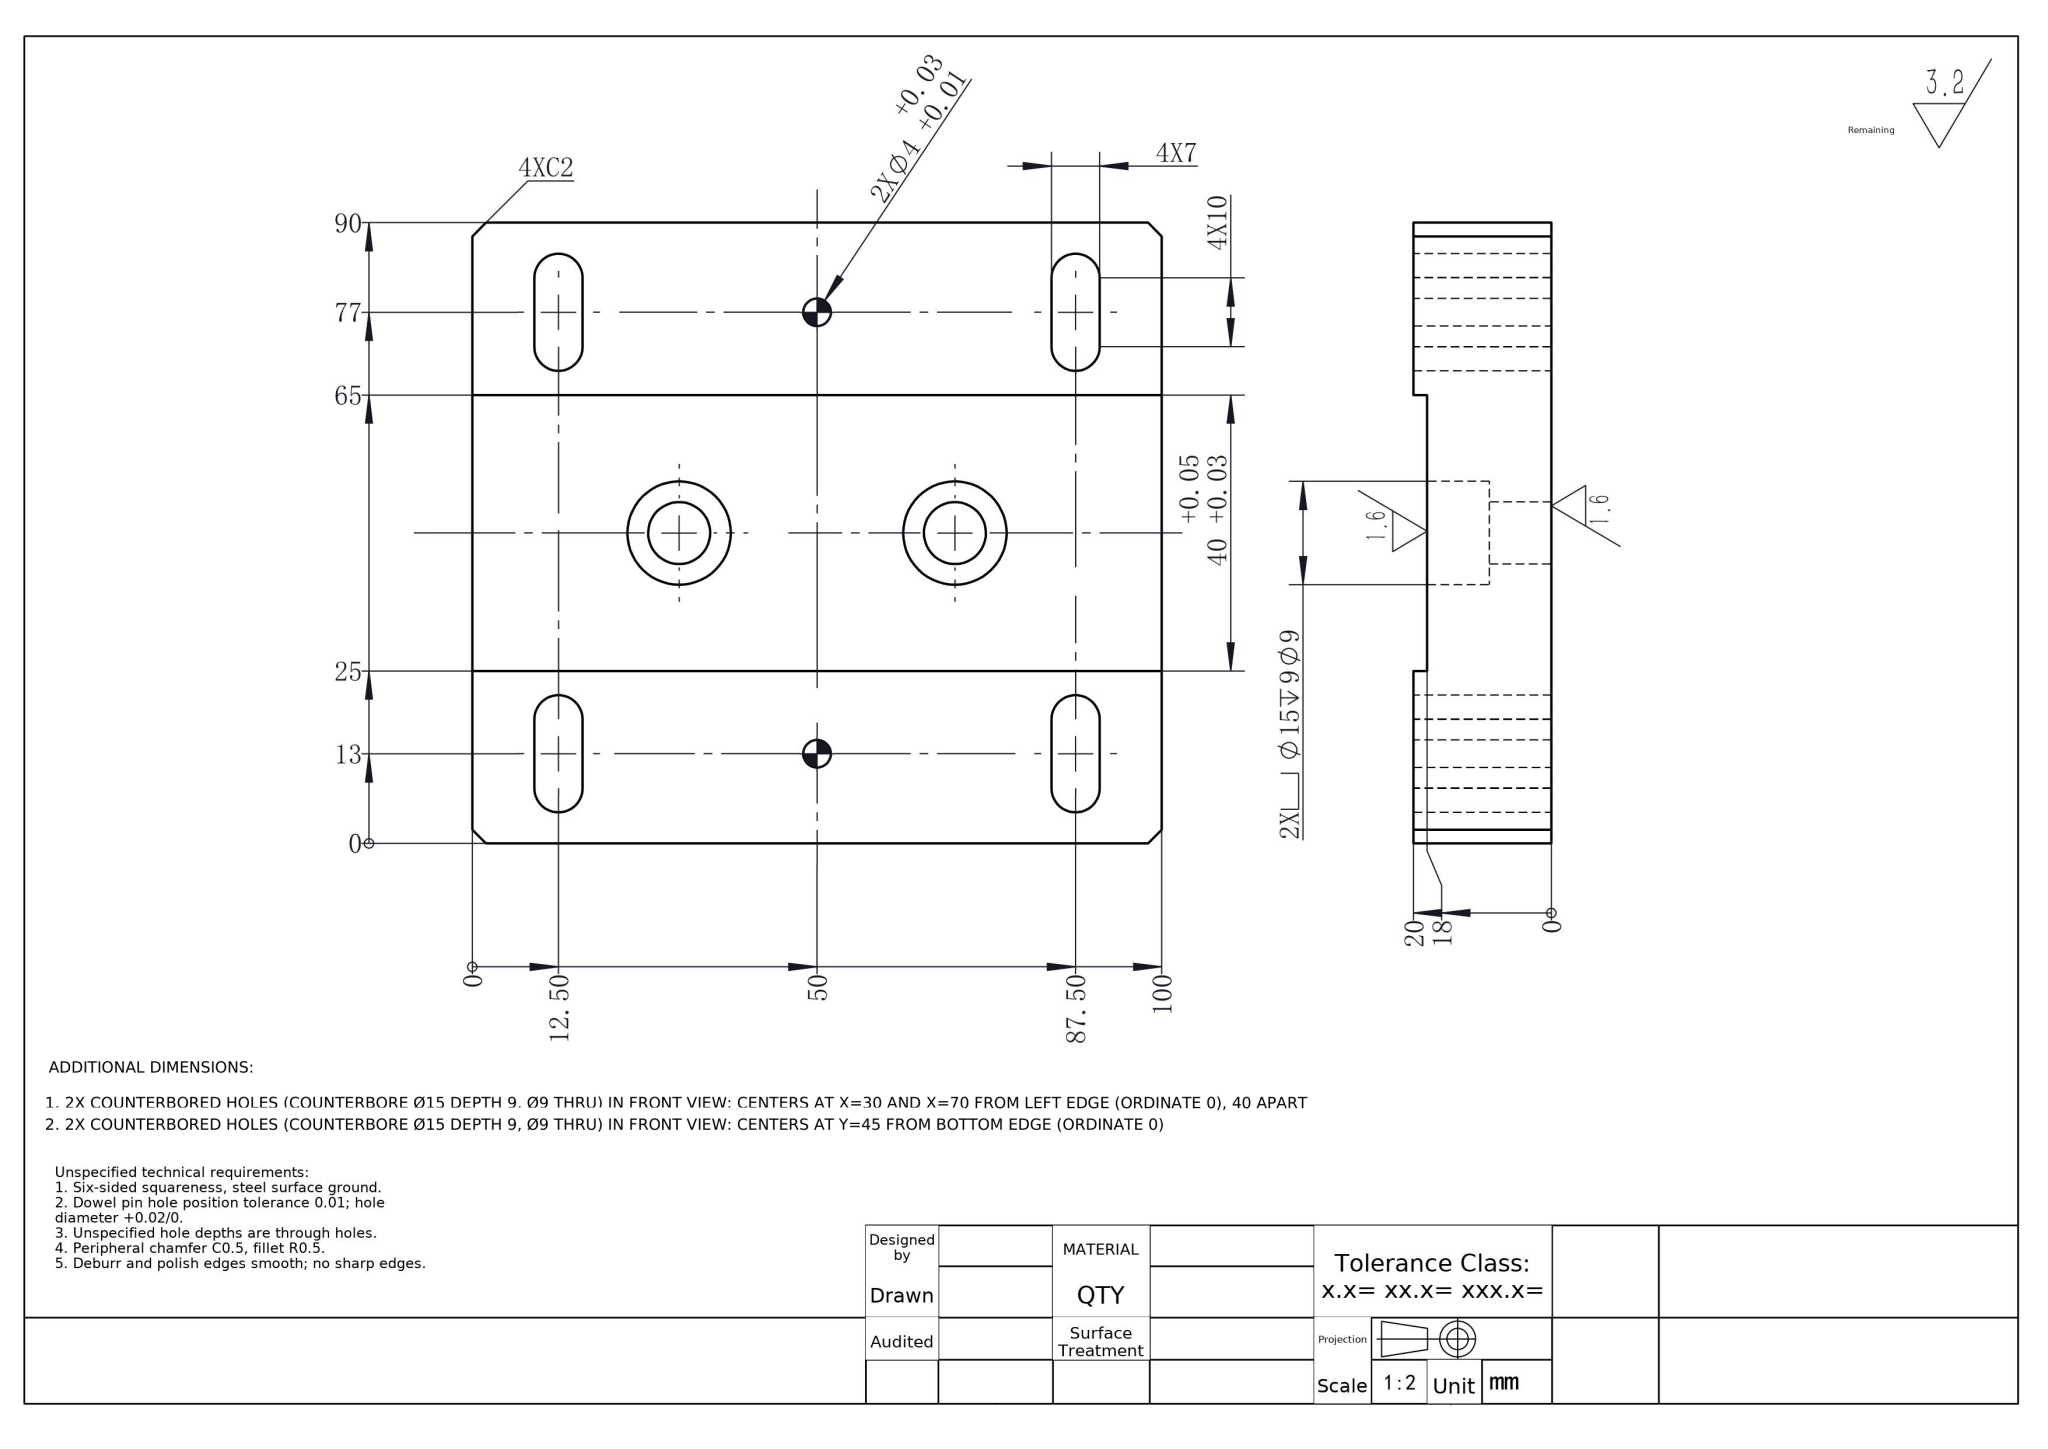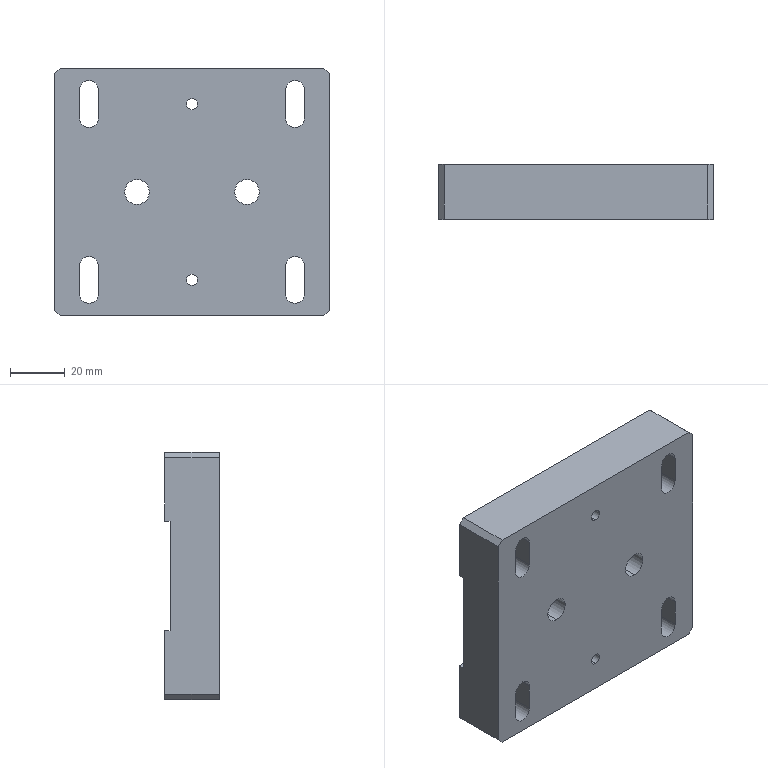Part | NX | mm | 1 solid | 48 faces | box 100 x 20 x 90 mm | volume 158333 mm3 | cylinder 24 | plane 24 | commonest cylinder face diameters 7 x12 4 x4 15 x4 9 x4